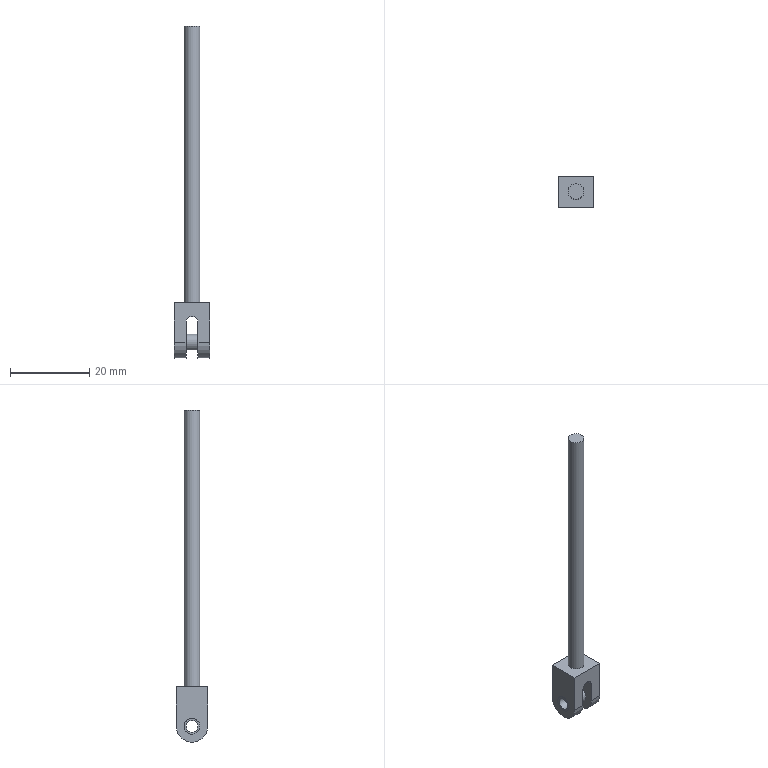Component | NX | 22C__27 | 2 solids | 18 faces | volume 1576 mm3 | plane 10 | cylinder 8 | commonest cylinder face diameters 4 x4 3 x2 8 x2